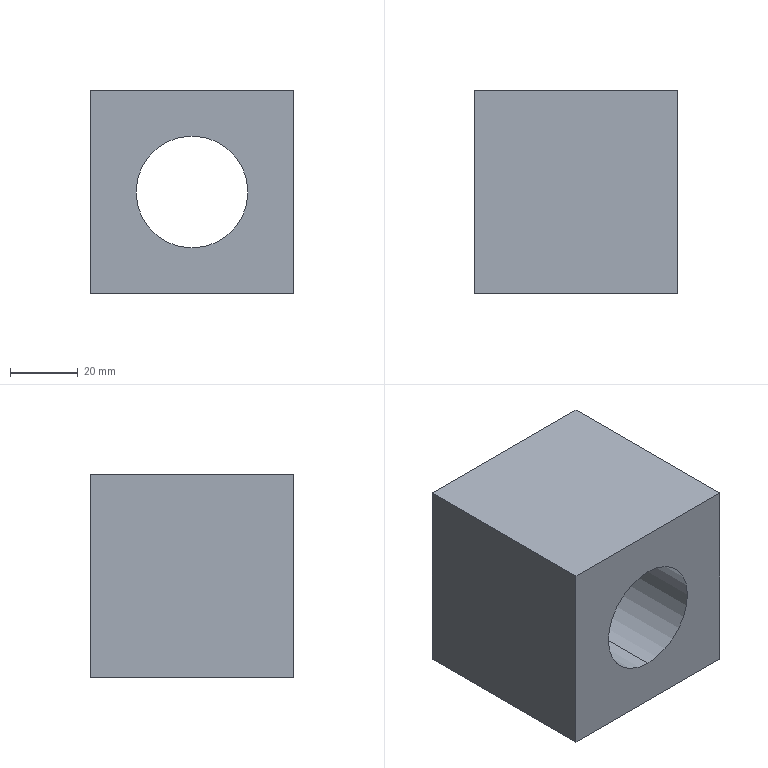Component | SolidWorks | JF21-80.1-1-3(_)-1-SOLID44-1 | 1 solid | 8 faces | box 60 x 60 x 60 mm | volume 164682 mm3 | plane 6 | cylinder 2 | commonest cylinder face diameters 33 x2
STEP:
#1=COLOUR_RGB('',0.7922,0.8196,0.9333);
#2=FILL_AREA_STYLE_COLOUR('',#1);
#3=FILL_AREA_STYLE('',(#2));
#4=SURFACE_STYLE_FILL_AREA(#3);
#5=SURFACE_SIDE_STYLE('',(#4));
#6=SURFACE_STYLE_USAGE(.BOTH.,#5);
#7=PRESENTATION_STYLE_ASSIGNMENT((#6));
#8=CARTESIAN_POINT('',(0.,-64.567,-10.689));
#9=VERTEX_POINT('',#8);
#10=CARTESIAN_POINT('',(0.,-64.567,-9.39));
#11=VERTEX_POINT('',#10);
#12=CARTESIAN_POINT('',(0.,-64.567,-10.039));
#13=DIRECTION('',(0.,1.,0.));
#14=DIRECTION('',(0.,0.,1.));
#15=AXIS2_PLACEMENT_3D('',#12,#13,#14);
#16=CIRCLE('',#15,0.6496);
#17=EDGE_CURVE('',#9,#11,#16,.T.);
#18=ORIENTED_EDGE('',*,*,#17,.F.);
#19=CARTESIAN_POINT('',(0.,-62.205,-10.689));
#20=VERTEX_POINT('',#19);
#21=CARTESIAN_POINT('',(0.,-62.205,-10.689));
#22=DIRECTION('',(0.,1.,0.));
#23=VECTOR('',#22,39.37);
#24=LINE('',#21,#23);
#25=EDGE_CURVE('',#9,#20,#24,.T.);
#26=ORIENTED_EDGE('',*,*,#25,.T.);
#27=CARTESIAN_POINT('',(0.,-62.205,-9.39));
#28=VERTEX_POINT('',#27);
#29=CARTESIAN_POINT('',(0.,-62.205,-10.039));
#30=DIRECTION('',(0.,1.,0.));
#31=DIRECTION('',(0.,0.,1.));
#32=AXIS2_PLACEMENT_3D('',#29,#30,#31);
#33=CIRCLE('',#32,0.6496);
#34=EDGE_CURVE('',#20,#28,#33,.T.);
#35=ORIENTED_EDGE('',*,*,#34,.T.);
#36=CARTESIAN_POINT('',(0.,-62.205,-9.39));
#37=DIRECTION('',(0.,1.,0.));
#38=VECTOR('',#37,39.37);
#39=LINE('',#36,#38);
#40=EDGE_CURVE('',#11,#28,#39,.T.);
#41=ORIENTED_EDGE('',*,*,#40,.F.);
#42=EDGE_LOOP('',(#18,#26,#35,#41));
#43=FACE_OUTER_BOUND('',#42,.T.);
#44=CARTESIAN_POINT('',(0.,-62.205,-10.039));
#45=DIRECTION('',(0.,1.,0.));
#46=DIRECTION('',(0.,0.,-1.));
#47=AXIS2_PLACEMENT_3D('',#44,#45,#46);
#48=CYLINDRICAL_SURFACE('',#47,0.6496);
#49=ADVANCED_FACE('',(#43),#48,.F.);
#50=CARTESIAN_POINT('',(1.181,-62.205,-8.858));
#51=VERTEX_POINT('',#50);
#52=CARTESIAN_POINT('',(1.181,-62.205,-11.22));
#53=VERTEX_POINT('',#52);
#54=CARTESIAN_POINT('',(1.181,-62.205,-8.858));
#55=DIRECTION('',(0.,0.,-1.));
#56=VECTOR('',#55,39.37);
#57=LINE('',#54,#56);
#58=EDGE_CURVE('',#51,#53,#57,.T.);
#59=ORIENTED_EDGE('',*,*,#58,.F.);
#60=CARTESIAN_POINT('',(1.181,-64.567,-8.858));
#61=VERTEX_POINT('',#60);
#62=CARTESIAN_POINT('',(1.181,-64.567,-8.858));
#63=DIRECTION('',(0.,1.,0.));
#64=VECTOR('',#63,39.37);
#65=LINE('',#62,#64);
#66=EDGE_CURVE('',#61,#51,#65,.T.);
#67=ORIENTED_EDGE('',*,*,#66,.F.);
#68=CARTESIAN_POINT('',(1.181,-64.567,-11.22));
#69=VERTEX_POINT('',#68);
#70=CARTESIAN_POINT('',(1.181,-64.567,-8.858));
#71=DIRECTION('',(0.,0.,-1.));
#72=VECTOR('',#71,39.37);
#73=LINE('',#70,#72);
#74=EDGE_CURVE('',#61,#69,#73,.T.);
#75=ORIENTED_EDGE('',*,*,#74,.T.);
#76=CARTESIAN_POINT('',(1.181,-64.567,-11.22));
#77=DIRECTION('',(0.,1.,0.));
#78=VECTOR('',#77,39.37);
#79=LINE('',#76,#78);
#80=EDGE_CURVE('',#69,#53,#79,.T.);
#81=ORIENTED_EDGE('',*,*,#80,.T.);
#82=EDGE_LOOP('',(#59,#67,#75,#81));
#83=FACE_OUTER_BOUND('',#82,.T.);
#84=CARTESIAN_POINT('',(1.181,-64.567,-8.858));
#85=DIRECTION('',(1.,0.,0.));
#86=DIRECTION('',(0.,0.,1.));
#87=AXIS2_PLACEMENT_3D('',#84,#85,#86);
#88=PLANE('',#87);
#89=ADVANCED_FACE('',(#83),#88,.T.);
#90=CARTESIAN_POINT('',(-1.181,-62.205,-8.858));
#91=VERTEX_POINT('',#90);
#92=CARTESIAN_POINT('',(1.181,-62.205,-8.858));
#93=DIRECTION('',(1.,0.,0.));
#94=VECTOR('',#93,39.37);
#95=LINE('',#92,#94);
#96=EDGE_CURVE('',#91,#51,#95,.T.);
#97=ORIENTED_EDGE('',*,*,#96,.F.);
#98=CARTESIAN_POINT('',(-1.181,-64.567,-8.858));
#99=VERTEX_POINT('',#98);
#100=CARTESIAN_POINT('',(-1.181,-64.567,-8.858));
#101=DIRECTION('',(0.,1.,0.));
#102=VECTOR('',#101,39.37);
#103=LINE('',#100,#102);
#104=EDGE_CURVE('',#99,#91,#103,.T.);
#105=ORIENTED_EDGE('',*,*,#104,.F.);
#106=CARTESIAN_POINT('',(1.181,-64.567,-8.858));
#107=DIRECTION('',(1.,0.,0.));
#108=VECTOR('',#107,39.37);
#109=LINE('',#106,#108);
#110=EDGE_CURVE('',#99,#61,#109,.T.);
#111=ORIENTED_EDGE('',*,*,#110,.T.);
#112=ORIENTED_EDGE('',*,*,#66,.T.);
#113=EDGE_LOOP('',(#97,#105,#111,#112));
#114=FACE_OUTER_BOUND('',#113,.T.);
#115=CARTESIAN_POINT('',(1.181,-64.567,-8.858));
#116=DIRECTION('',(0.,0.,1.));
#117=DIRECTION('',(-1.,0.,0.));
#118=AXIS2_PLACEMENT_3D('',#115,#116,#117);
#119=PLANE('',#118);
#120=ADVANCED_FACE('',(#114),#119,.T.);
#121=CARTESIAN_POINT('',(-1.181,-62.205,-11.22));
#122=VERTEX_POINT('',#121);
#123=CARTESIAN_POINT('',(-1.181,-62.205,-8.858));
#124=DIRECTION('',(0.,0.,1.));
#125=VECTOR('',#124,39.37);
#126=LINE('',#123,#125);
#127=EDGE_CURVE('',#122,#91,#126,.T.);
#128=ORIENTED_EDGE('',*,*,#127,.F.);
#129=CARTESIAN_POINT('',(-1.181,-64.567,-11.22));
#130=VERTEX_POINT('',#129);
#131=CARTESIAN_POINT('',(-1.181,-64.567,-11.22));
#132=DIRECTION('',(0.,1.,0.));
#133=VECTOR('',#132,39.37);
#134=LINE('',#131,#133);
#135=EDGE_CURVE('',#130,#122,#134,.T.);
#136=ORIENTED_EDGE('',*,*,#135,.F.);
#137=CARTESIAN_POINT('',(-1.181,-64.567,-8.858));
#138=DIRECTION('',(0.,0.,1.));
#139=VECTOR('',#138,39.37);
#140=LINE('',#137,#139);
#141=EDGE_CURVE('',#130,#99,#140,.T.);
#142=ORIENTED_EDGE('',*,*,#141,.T.);
#143=ORIENTED_EDGE('',*,*,#104,.T.);
#144=EDGE_LOOP('',(#128,#136,#142,#143));
#145=FACE_OUTER_BOUND('',#144,.T.);
#146=CARTESIAN_POINT('',(-1.181,-64.567,-8.858));
#147=DIRECTION('',(-1.,0.,0.));
#148=DIRECTION('',(-0.,0.,-1.));
#149=AXIS2_PLACEMENT_3D('',#146,#147,#148);
#150=PLANE('',#149);
#151=ADVANCED_FACE('',(#145),#150,.T.);
#152=CARTESIAN_POINT('',(1.181,-62.205,-11.22));
#153=DIRECTION('',(-1.,0.,0.));
#154=VECTOR('',#153,39.37);
#155=LINE('',#152,#154);
#156=EDGE_CURVE('',#53,#122,#155,.T.);
#157=ORIENTED_EDGE('',*,*,#156,.F.);
#158=ORIENTED_EDGE('',*,*,#80,.F.);
#159=CARTESIAN_POINT('',(1.181,-64.567,-11.22));
#160=DIRECTION('',(-1.,0.,0.));
#161=VECTOR('',#160,39.37);
#162=LINE('',#159,#161);
#163=EDGE_CURVE('',#69,#130,#162,.T.);
#164=ORIENTED_EDGE('',*,*,#163,.T.);
#165=ORIENTED_EDGE('',*,*,#135,.T.);
#166=EDGE_LOOP('',(#157,#158,#164,#165));
#167=FACE_OUTER_BOUND('',#166,.T.);
#168=CARTESIAN_POINT('',(1.181,-64.567,-11.22));
#169=DIRECTION('',(-0.,0.,-1.));
#170=DIRECTION('',(1.,0.,-0.));
#171=AXIS2_PLACEMENT_3D('',#168,#169,#170);
#172=PLANE('',#171);
#173=ADVANCED_FACE('',(#167),#172,.T.);
#174=CARTESIAN_POINT('',(0.,-64.567,-10.039));
#175=DIRECTION('',(0.,1.,0.));
#176=DIRECTION('',(0.,0.,1.));
#177=AXIS2_PLACEMENT_3D('',#174,#175,#176);
#178=CIRCLE('',#177,0.6496);
#179=EDGE_CURVE('',#11,#9,#178,.T.);
#180=ORIENTED_EDGE('',*,*,#179,.T.);
#181=ORIENTED_EDGE('',*,*,#17,.T.);
#182=EDGE_LOOP('',(#180,#181));
#183=FACE_BOUND('',#182,.T.);
#184=ORIENTED_EDGE('',*,*,#74,.F.);
#185=ORIENTED_EDGE('',*,*,#110,.F.);
#186=ORIENTED_EDGE('',*,*,#141,.F.);
#187=ORIENTED_EDGE('',*,*,#163,.F.);
#188=EDGE_LOOP('',(#184,#185,#186,#187));
#189=FACE_OUTER_BOUND('',#188,.T.);
#190=CARTESIAN_POINT('',(1.181,-64.567,-11.22));
#191=DIRECTION('',(0.,1.,0.));
#192=DIRECTION('',(0.,0.,-1.));
#193=AXIS2_PLACEMENT_3D('',#190,#191,#192);
#194=PLANE('',#193);
#195=ADVANCED_FACE('',(#183,#189),#194,.F.);
#196=CARTESIAN_POINT('',(0.,-62.205,-10.039));
#197=DIRECTION('',(0.,1.,0.));
#198=DIRECTION('',(0.,0.,1.));
#199=AXIS2_PLACEMENT_3D('',#196,#197,#198);
#200=CIRCLE('',#199,0.6496);
#201=EDGE_CURVE('',#28,#20,#200,.T.);
#202=ORIENTED_EDGE('',*,*,#201,.F.);
#203=ORIENTED_EDGE('',*,*,#34,.F.);
#204=EDGE_LOOP('',(#202,#203));
#205=FACE_BOUND('',#204,.T.);
#206=ORIENTED_EDGE('',*,*,#58,.T.);
#207=ORIENTED_EDGE('',*,*,#156,.T.);
#208=ORIENTED_EDGE('',*,*,#127,.T.);
#209=ORIENTED_EDGE('',*,*,#96,.T.);
#210=EDGE_LOOP('',(#206,#207,#208,#209));
#211=FACE_OUTER_BOUND('',#210,.T.);
#212=CARTESIAN_POINT('',(1.181,-62.205,-11.22));
#213=DIRECTION('',(0.,1.,0.));
#214=DIRECTION('',(0.,0.,-1.));
#215=AXIS2_PLACEMENT_3D('',#212,#213,#214);
#216=PLANE('',#215);
#217=ADVANCED_FACE('',(#205,#211),#216,.T.);
#218=ORIENTED_EDGE('',*,*,#25,.F.);
#219=ORIENTED_EDGE('',*,*,#179,.F.);
#220=ORIENTED_EDGE('',*,*,#40,.T.);
#221=ORIENTED_EDGE('',*,*,#201,.T.);
#222=EDGE_LOOP('',(#218,#219,#220,#221));
#223=FACE_OUTER_BOUND('',#222,.T.);
#224=CARTESIAN_POINT('',(0.,-62.205,-10.039));
#225=DIRECTION('',(0.,1.,0.));
#226=DIRECTION('',(0.,0.,-1.));
#227=AXIS2_PLACEMENT_3D('',#224,#225,#226);
#228=CYLINDRICAL_SURFACE('',#227,0.6496);
#229=ADVANCED_FACE('',(#223),#228,.F.);
#230=CLOSED_SHELL('',(#49,#89,#120,#151,#173,#195,#217,#229));
#231=MANIFOLD_SOLID_BREP('',#230);
#232=STYLED_ITEM('',(#7),#231);
#233=(LENGTH_UNIT()NAMED_UNIT(*)SI_UNIT($,.METRE.));
#234=LENGTH_MEASURE_WITH_UNIT(LENGTH_MEASURE(0.0254),#233);
#235=DIMENSIONAL_EXPONENTS(1.,0.,0.,0.,0.,0.,0.);
#236=(CONVERSION_BASED_UNIT('',#234)LENGTH_UNIT()NAMED_UNIT(#235));
#237=UNCERTAINTY_MEASURE_WITH_UNIT(LENGTH_MEASURE(0.00001),#236,'','');
#238=(NAMED_UNIT(*)PLANE_ANGLE_UNIT()SI_UNIT($,.RADIAN.));
#239=(NAMED_UNIT(*)SI_UNIT($,.STERADIAN.)SOLID_ANGLE_UNIT());
#240=(GEOMETRIC_REPRESENTATION_CONTEXT(3)GLOBAL_UNCERTAINTY_ASSIGNED_CONTEXT((#237))GLOBAL_UNIT_ASSIGNED_CONTEXT((#236,#238,#239))REPRESENTATION_CONTEXT('',''));
#241=MECHANICAL_DESIGN_GEOMETRIC_PRESENTATION_REPRESENTATION('',(#232),#240);
#242=PRESENTATION_LAYER_ASSIGNMENT('','',(#232));
#243=CARTESIAN_POINT('',(0.,0.,0.));
#244=DIRECTION('',(0.,0.,1.));
#245=DIRECTION('',(1.,0.,0.));
#246=AXIS2_PLACEMENT_3D('',#243,#244,#245);
#247=(LENGTH_UNIT()NAMED_UNIT(*)SI_UNIT($,.METRE.));
#248=LENGTH_MEASURE_WITH_UNIT(LENGTH_MEASURE(0.0254),#247);
#249=DIMENSIONAL_EXPONENTS(1.,0.,0.,0.,0.,0.,0.);
#250=(CONVERSION_BASED_UNIT('',#248)LENGTH_UNIT()NAMED_UNIT(#249));
#251=UNCERTAINTY_MEASURE_WITH_UNIT(LENGTH_MEASURE(0.00001),#250,'','');
#252=(NAMED_UNIT(*)PLANE_ANGLE_UNIT()SI_UNIT($,.RADIAN.));
#253=(NAMED_UNIT(*)SI_UNIT($,.STERADIAN.)SOLID_ANGLE_UNIT());
#254=(GEOMETRIC_REPRESENTATION_CONTEXT(3)GLOBAL_UNCERTAINTY_ASSIGNED_CONTEXT((#251))GLOBAL_UNIT_ASSIGNED_CONTEXT((#250,#252,#253))REPRESENTATION_CONTEXT('',''));
#255=ADVANCED_BREP_SHAPE_REPRESENTATION('',(#231,#246),#254);